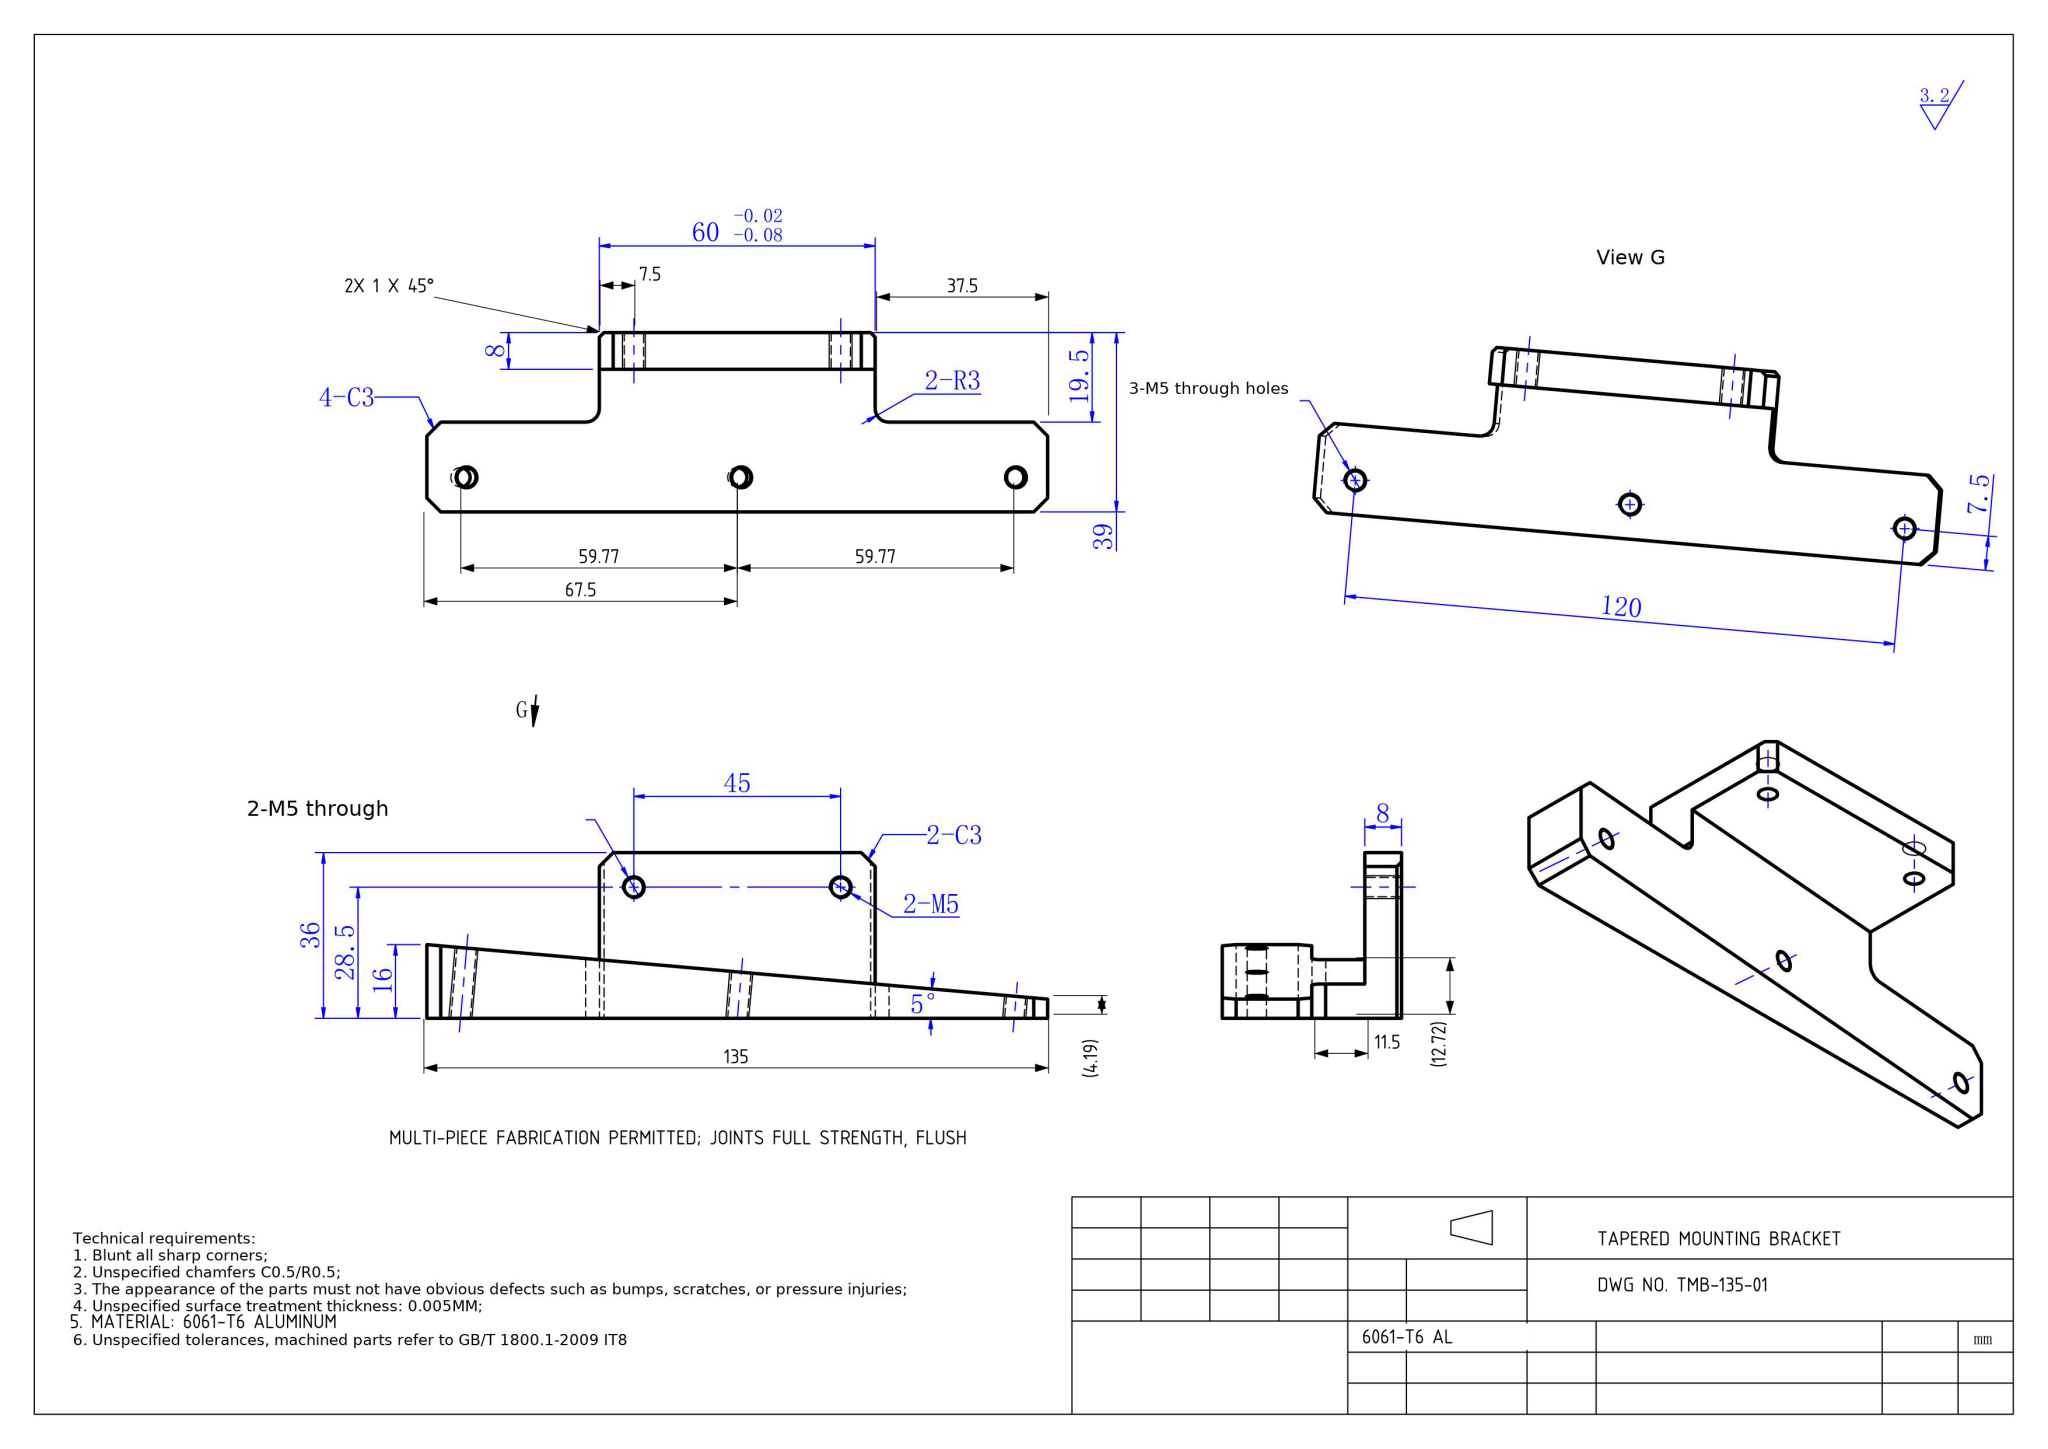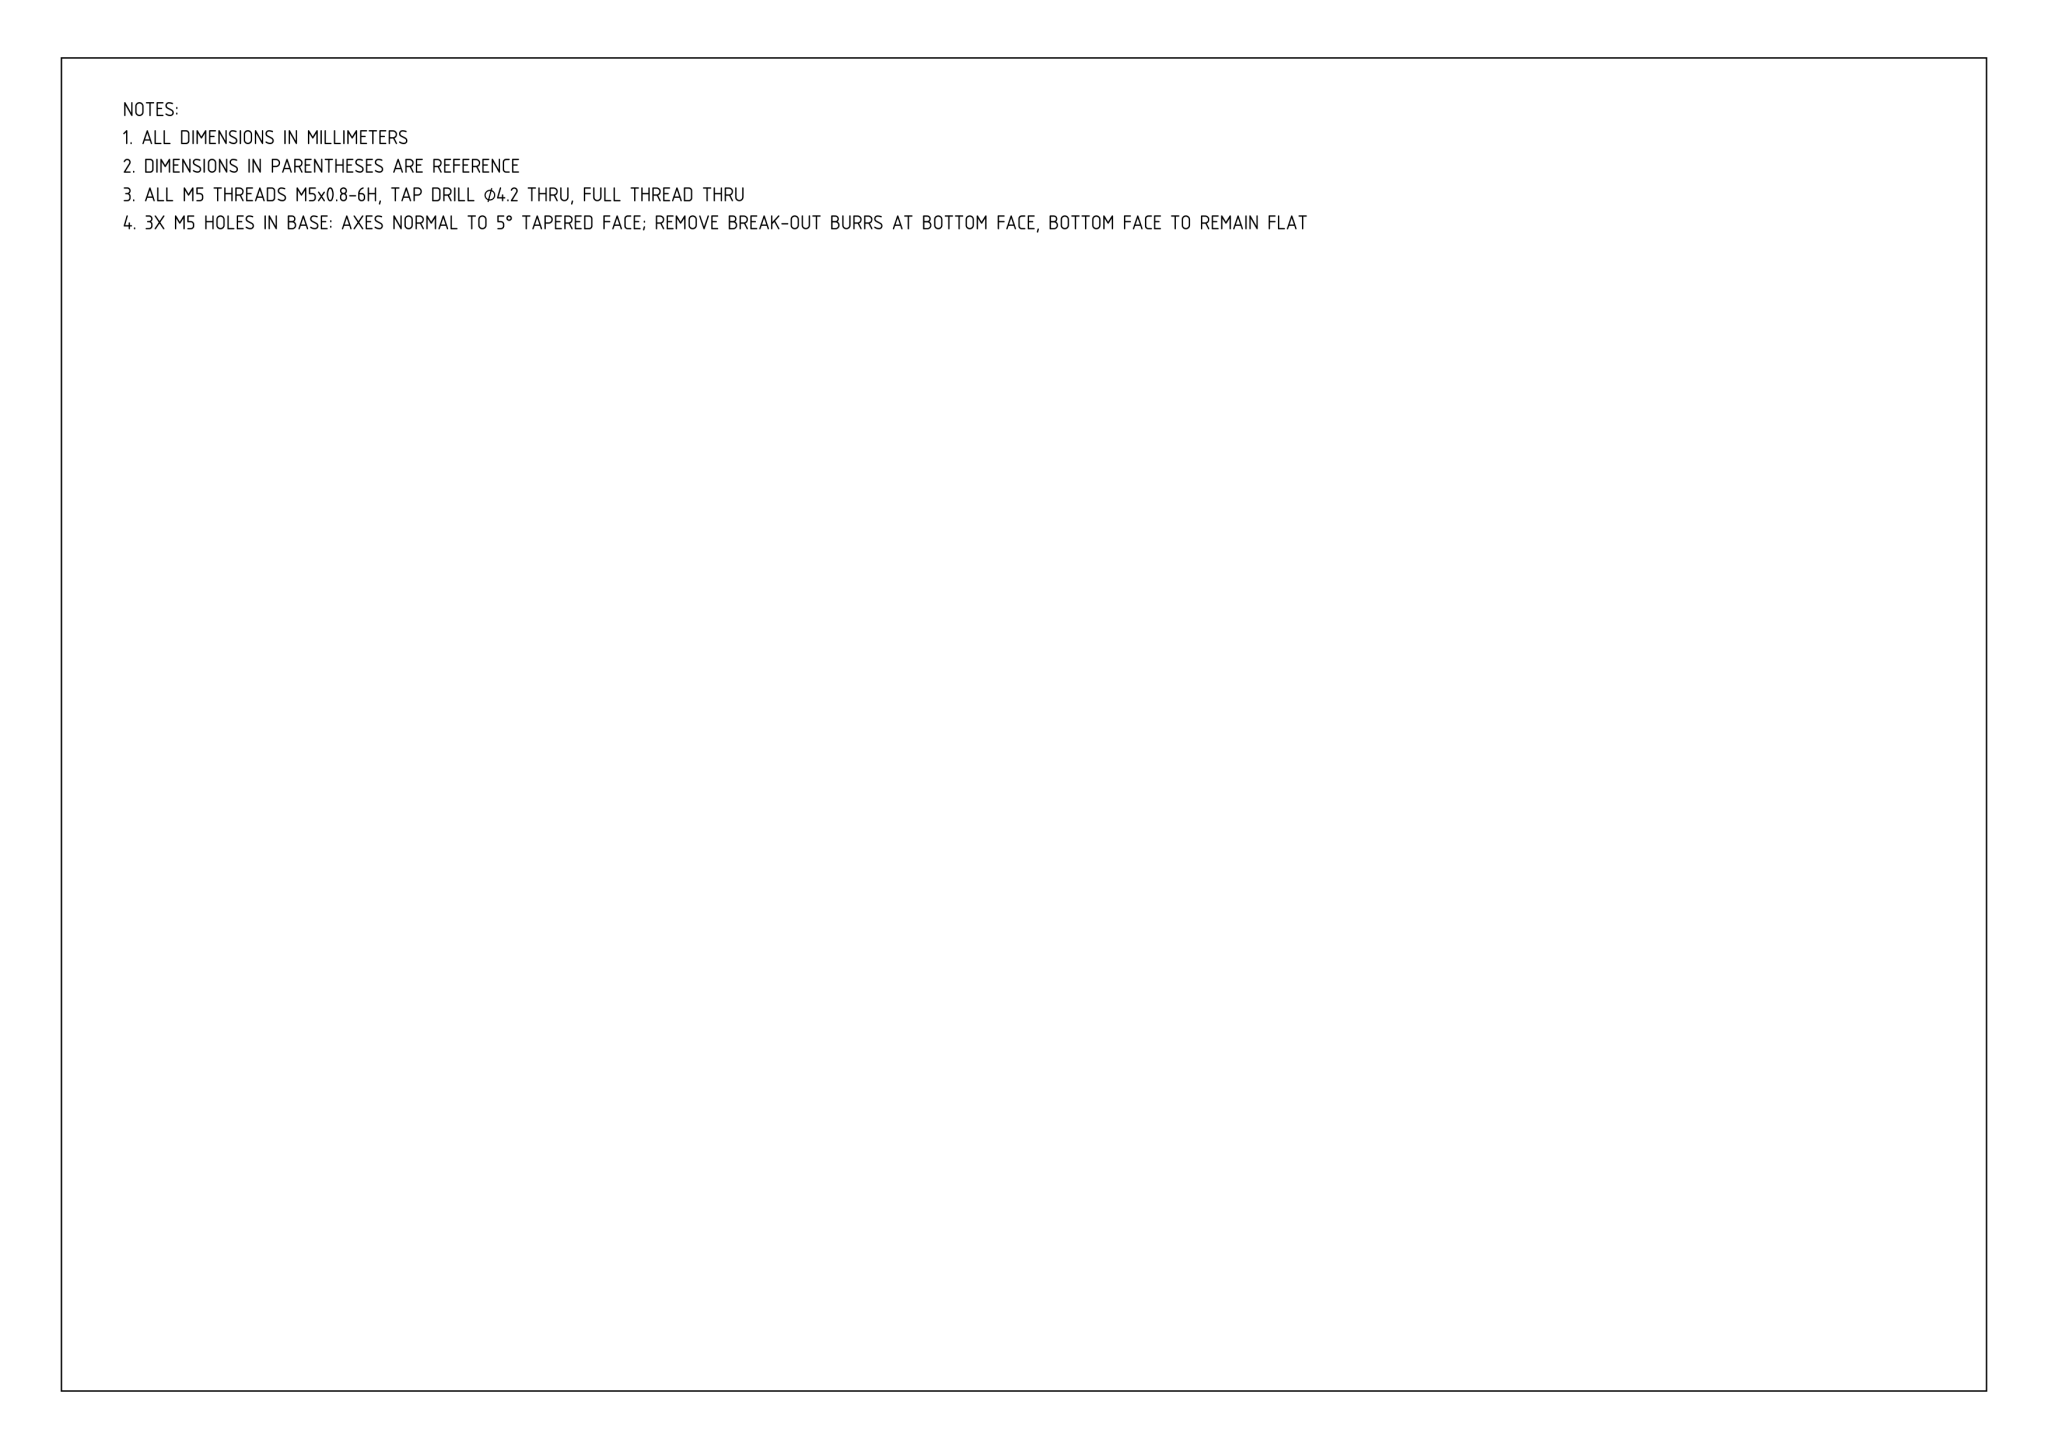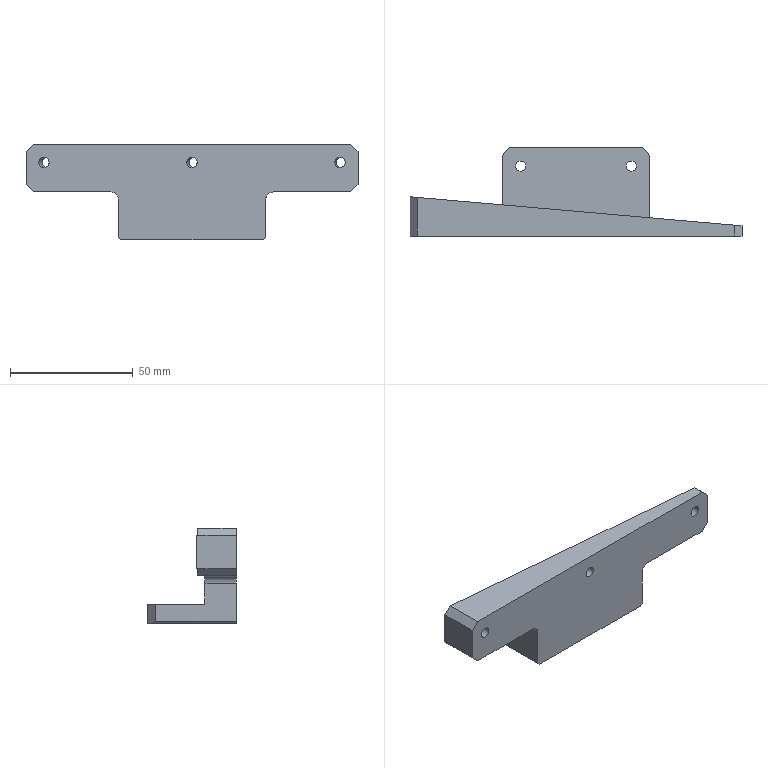Part | NX | mm | 1 solid | 32 faces | box 135 x 36 x 39 mm | volume 49931 mm3 | plane 20 | cylinder 12 | commonest cylinder face diameters 4.2 x10 6 x2